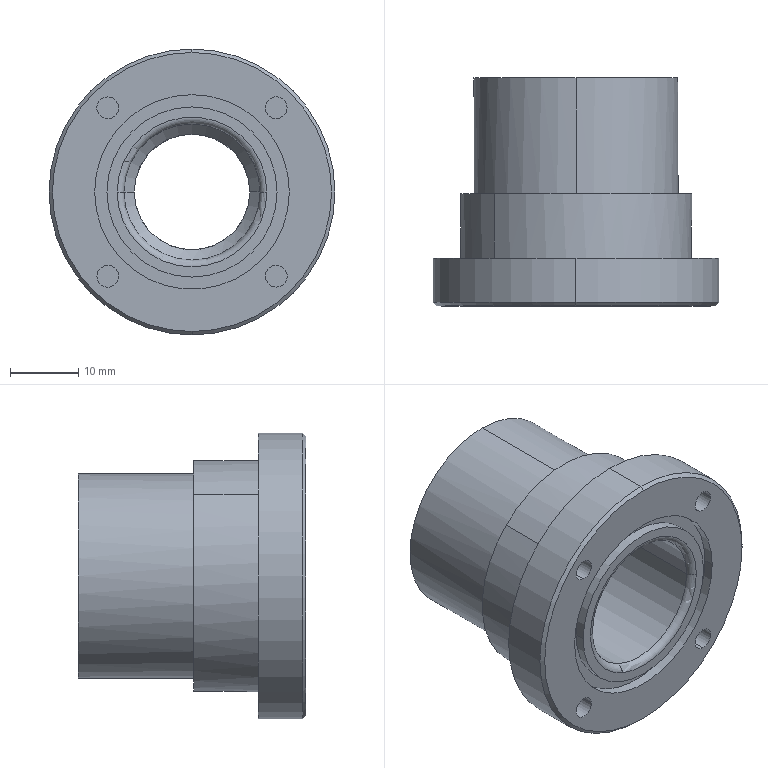CAM job | Mastercam | mm | 8 operations | part box 42 x 33.5 x 42
1. Drill/Counterbore | 7 - 4 倒角刀
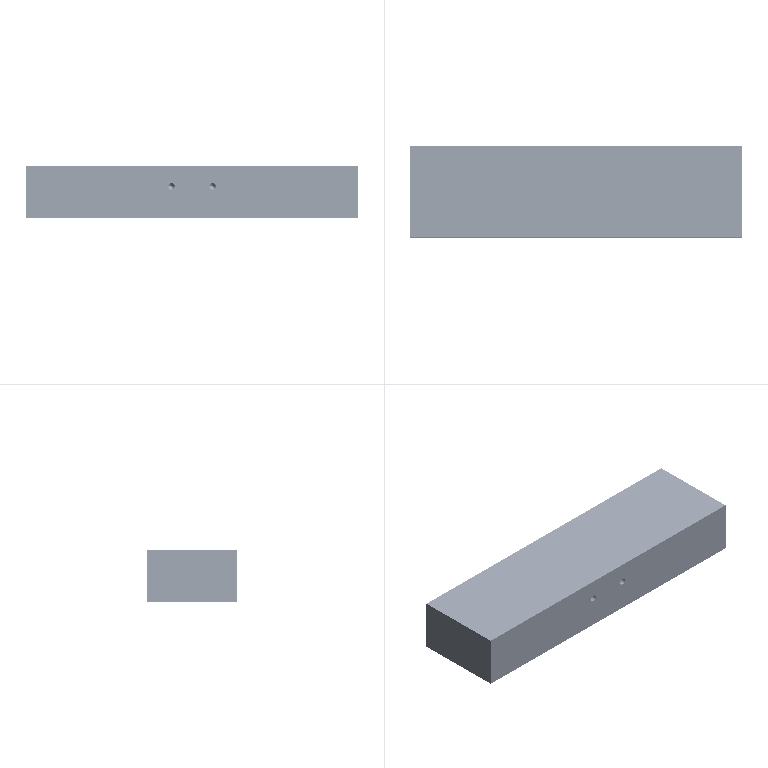2. Peck Drill | 1 - 3.4 钻头
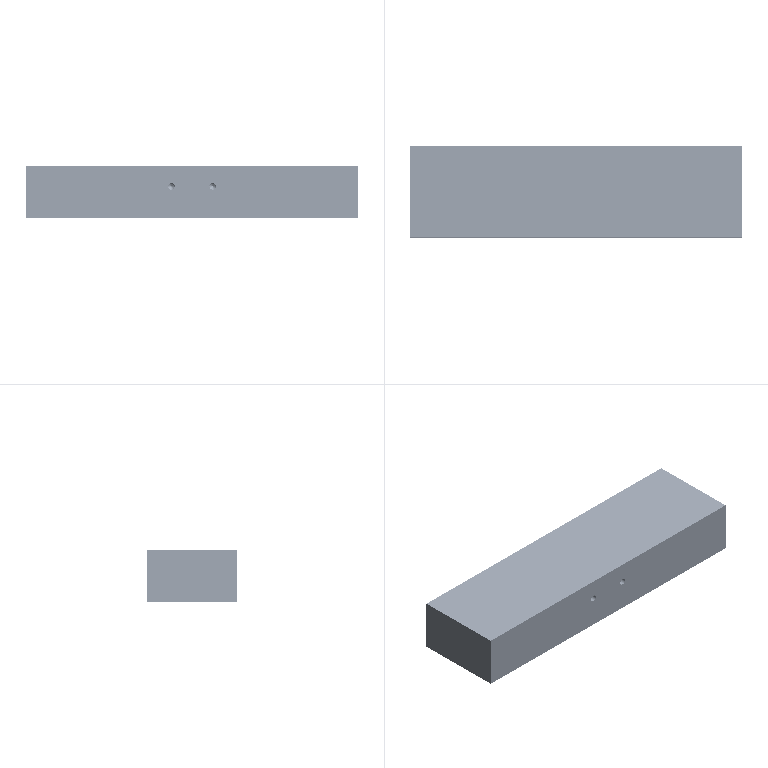3. Contour (2D chamfer) | 7 - 4 倒角刀
4. Drill/Counterbore | 7 - 4 倒角刀
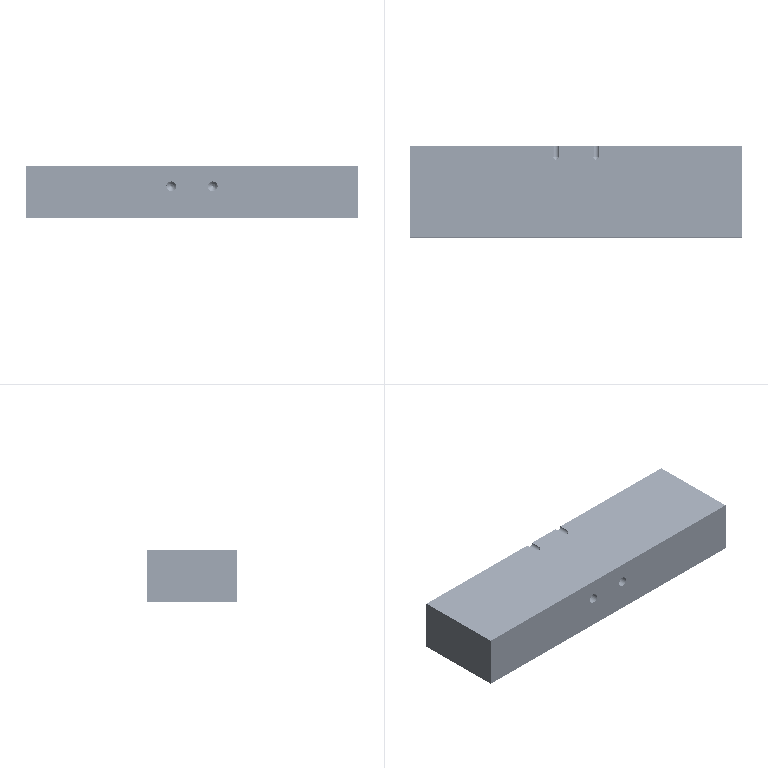5. Facing | 20 - 63 平铣刀
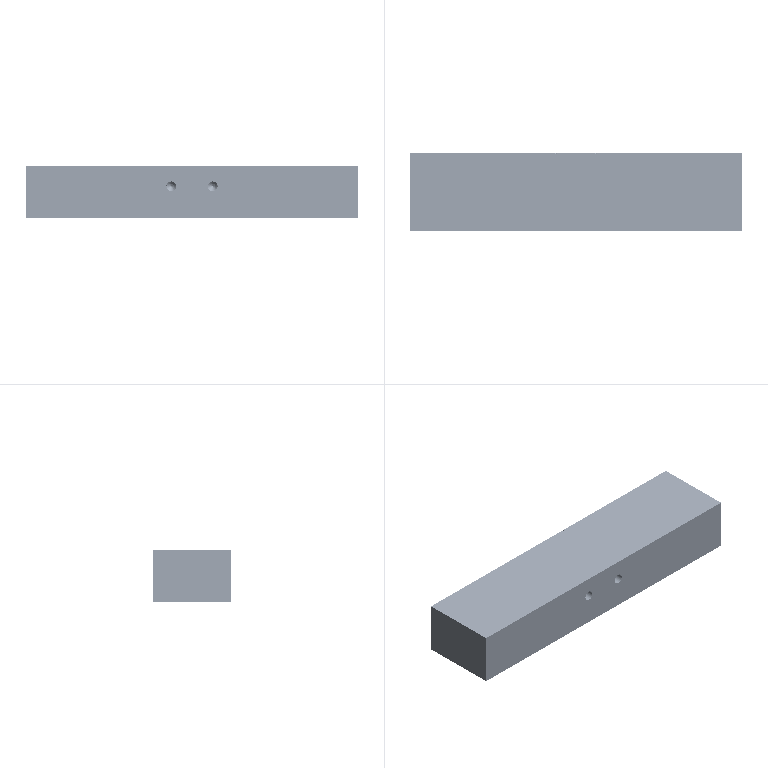6. 2D High Speed (2D Area Mill) | 6 - 6 平铣刀
7. Contour (2D) | 6 - 6 平铣刀
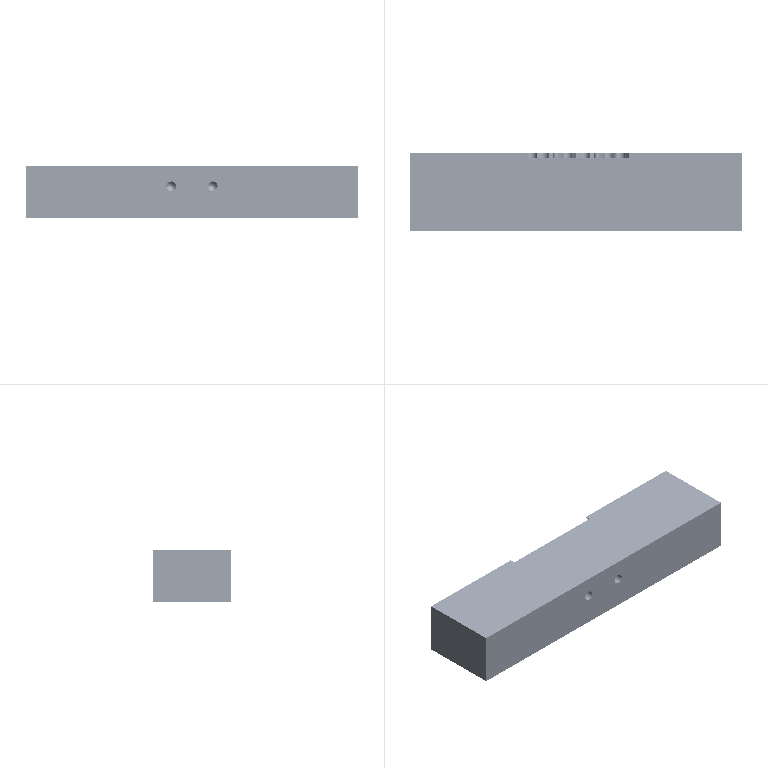8. Contour (2D chamfer) | 7 - 4 倒角刀